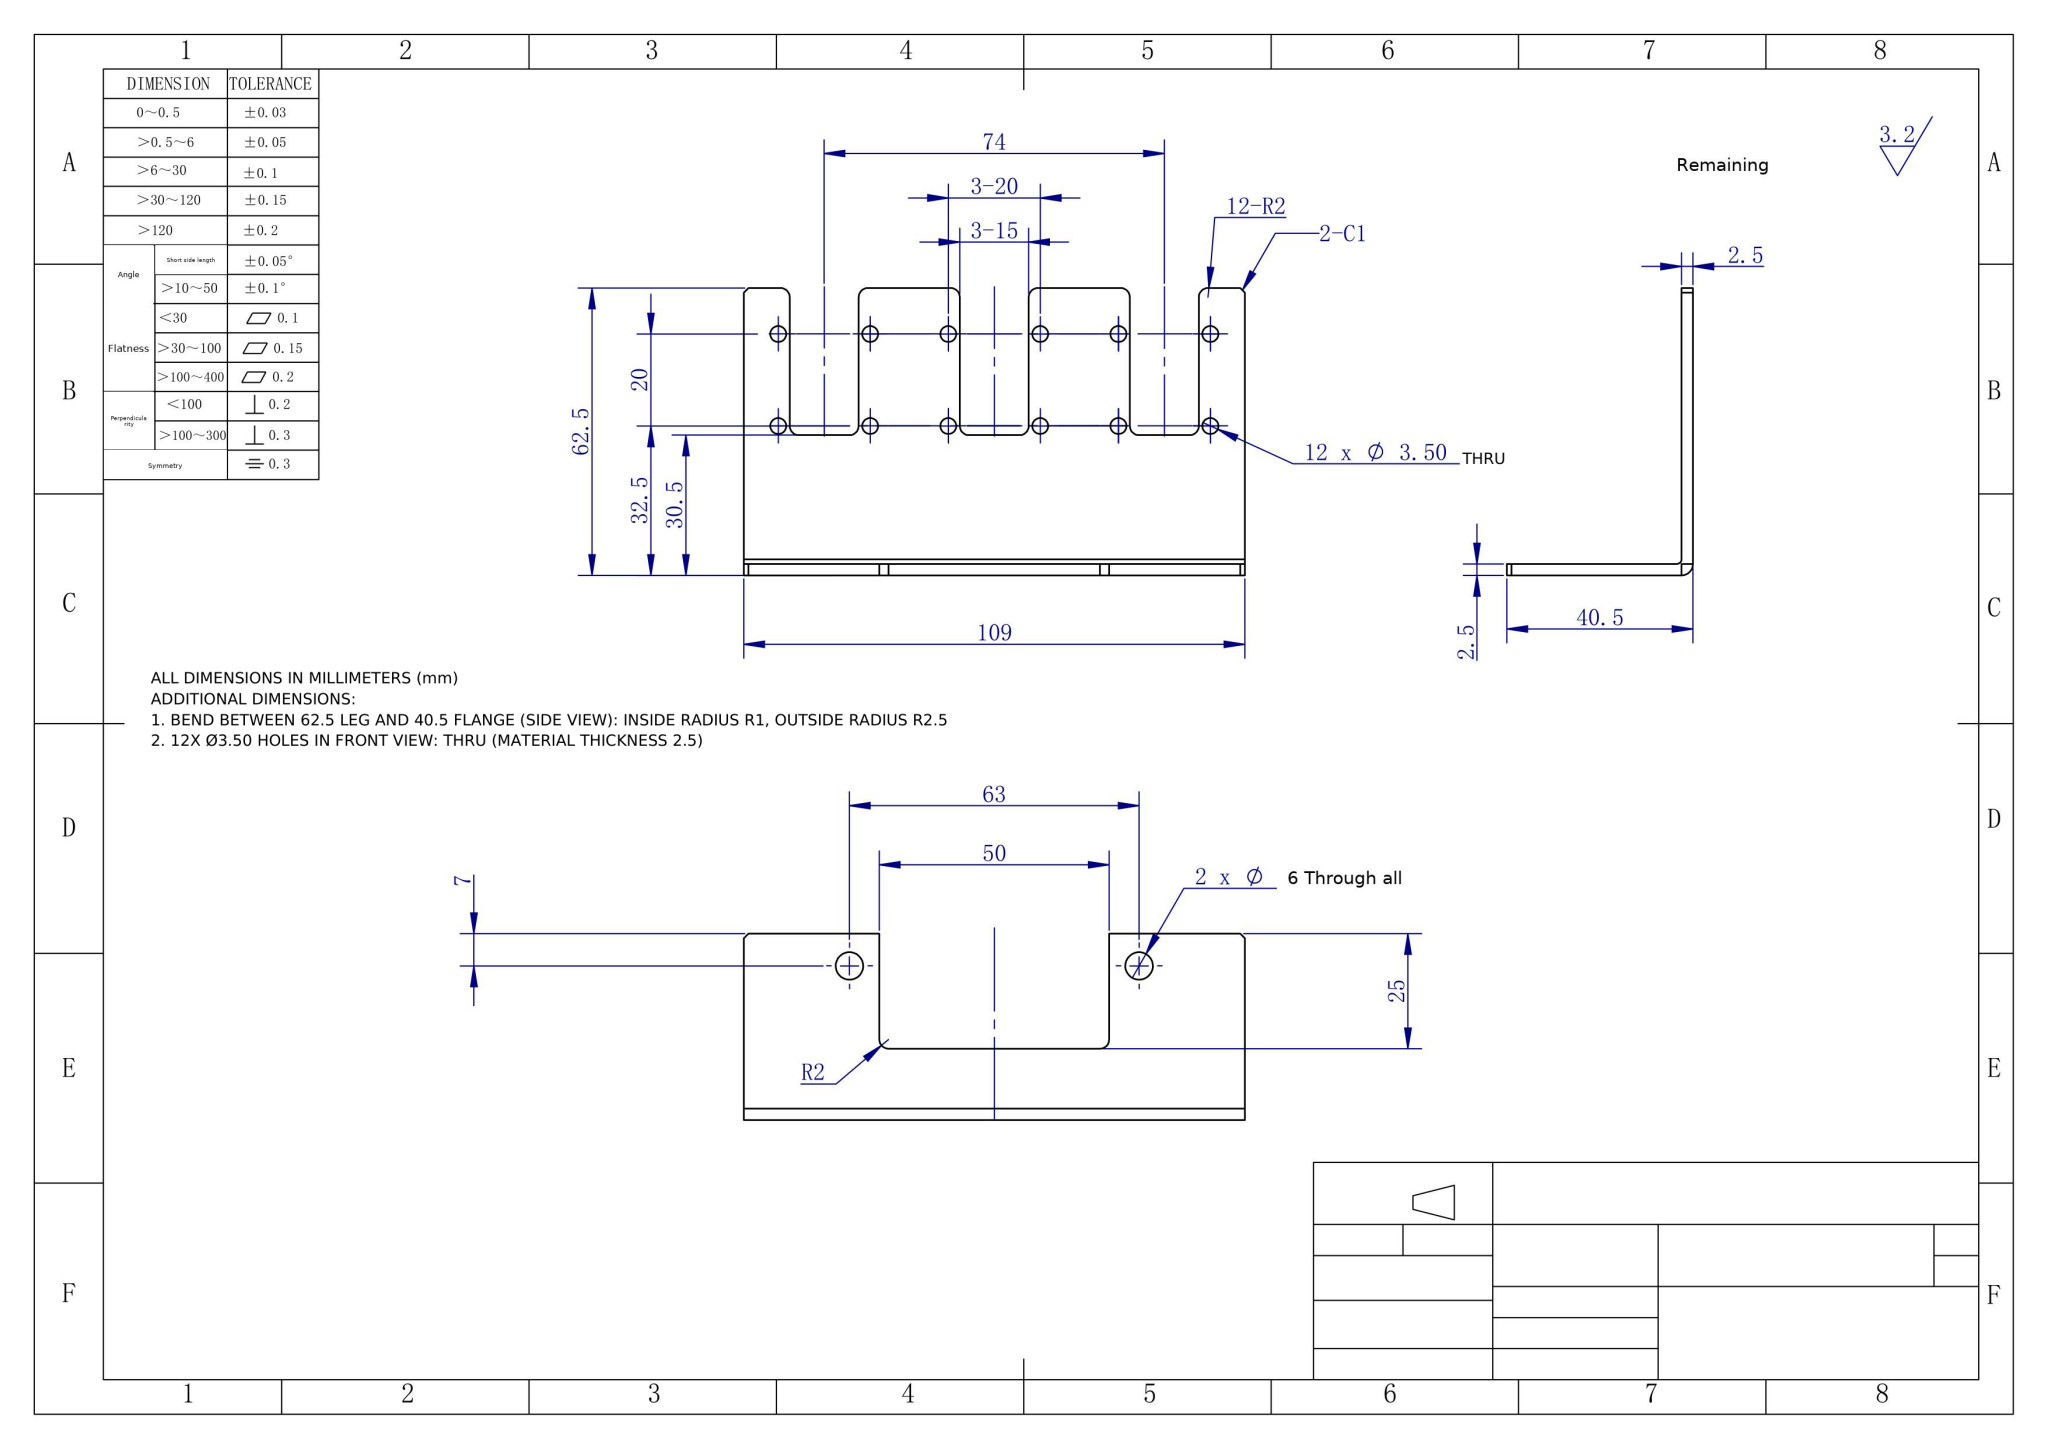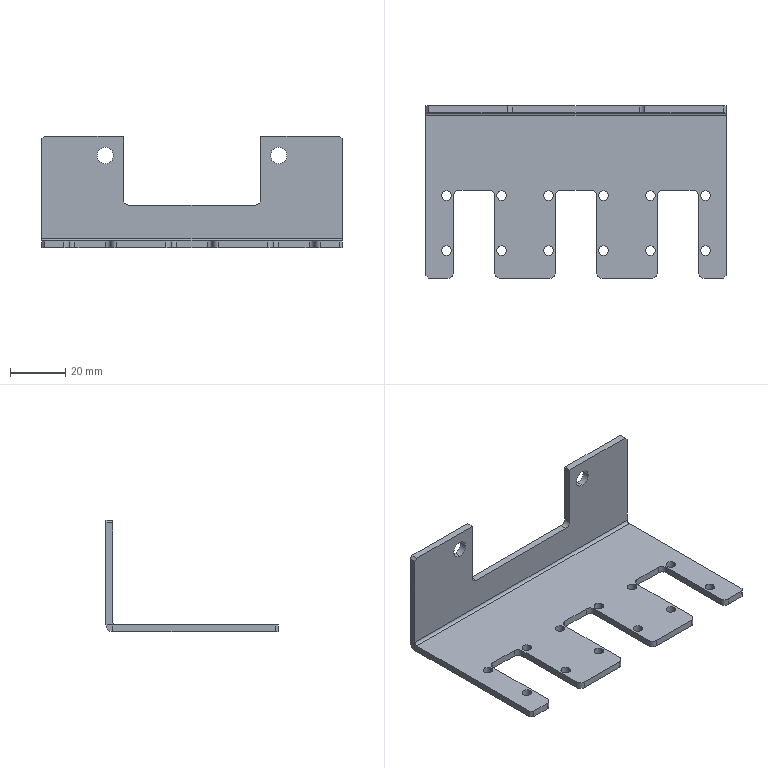Part | NX | mm | 1 solid | 74 faces | box 109 x 62.5 x 40.5 mm | volume 20108 mm3 | cylinder 44 | plane 30 | commonest cylinder face diameters 3.5 x24 4 x14 6 x4 5 x1 2 x1